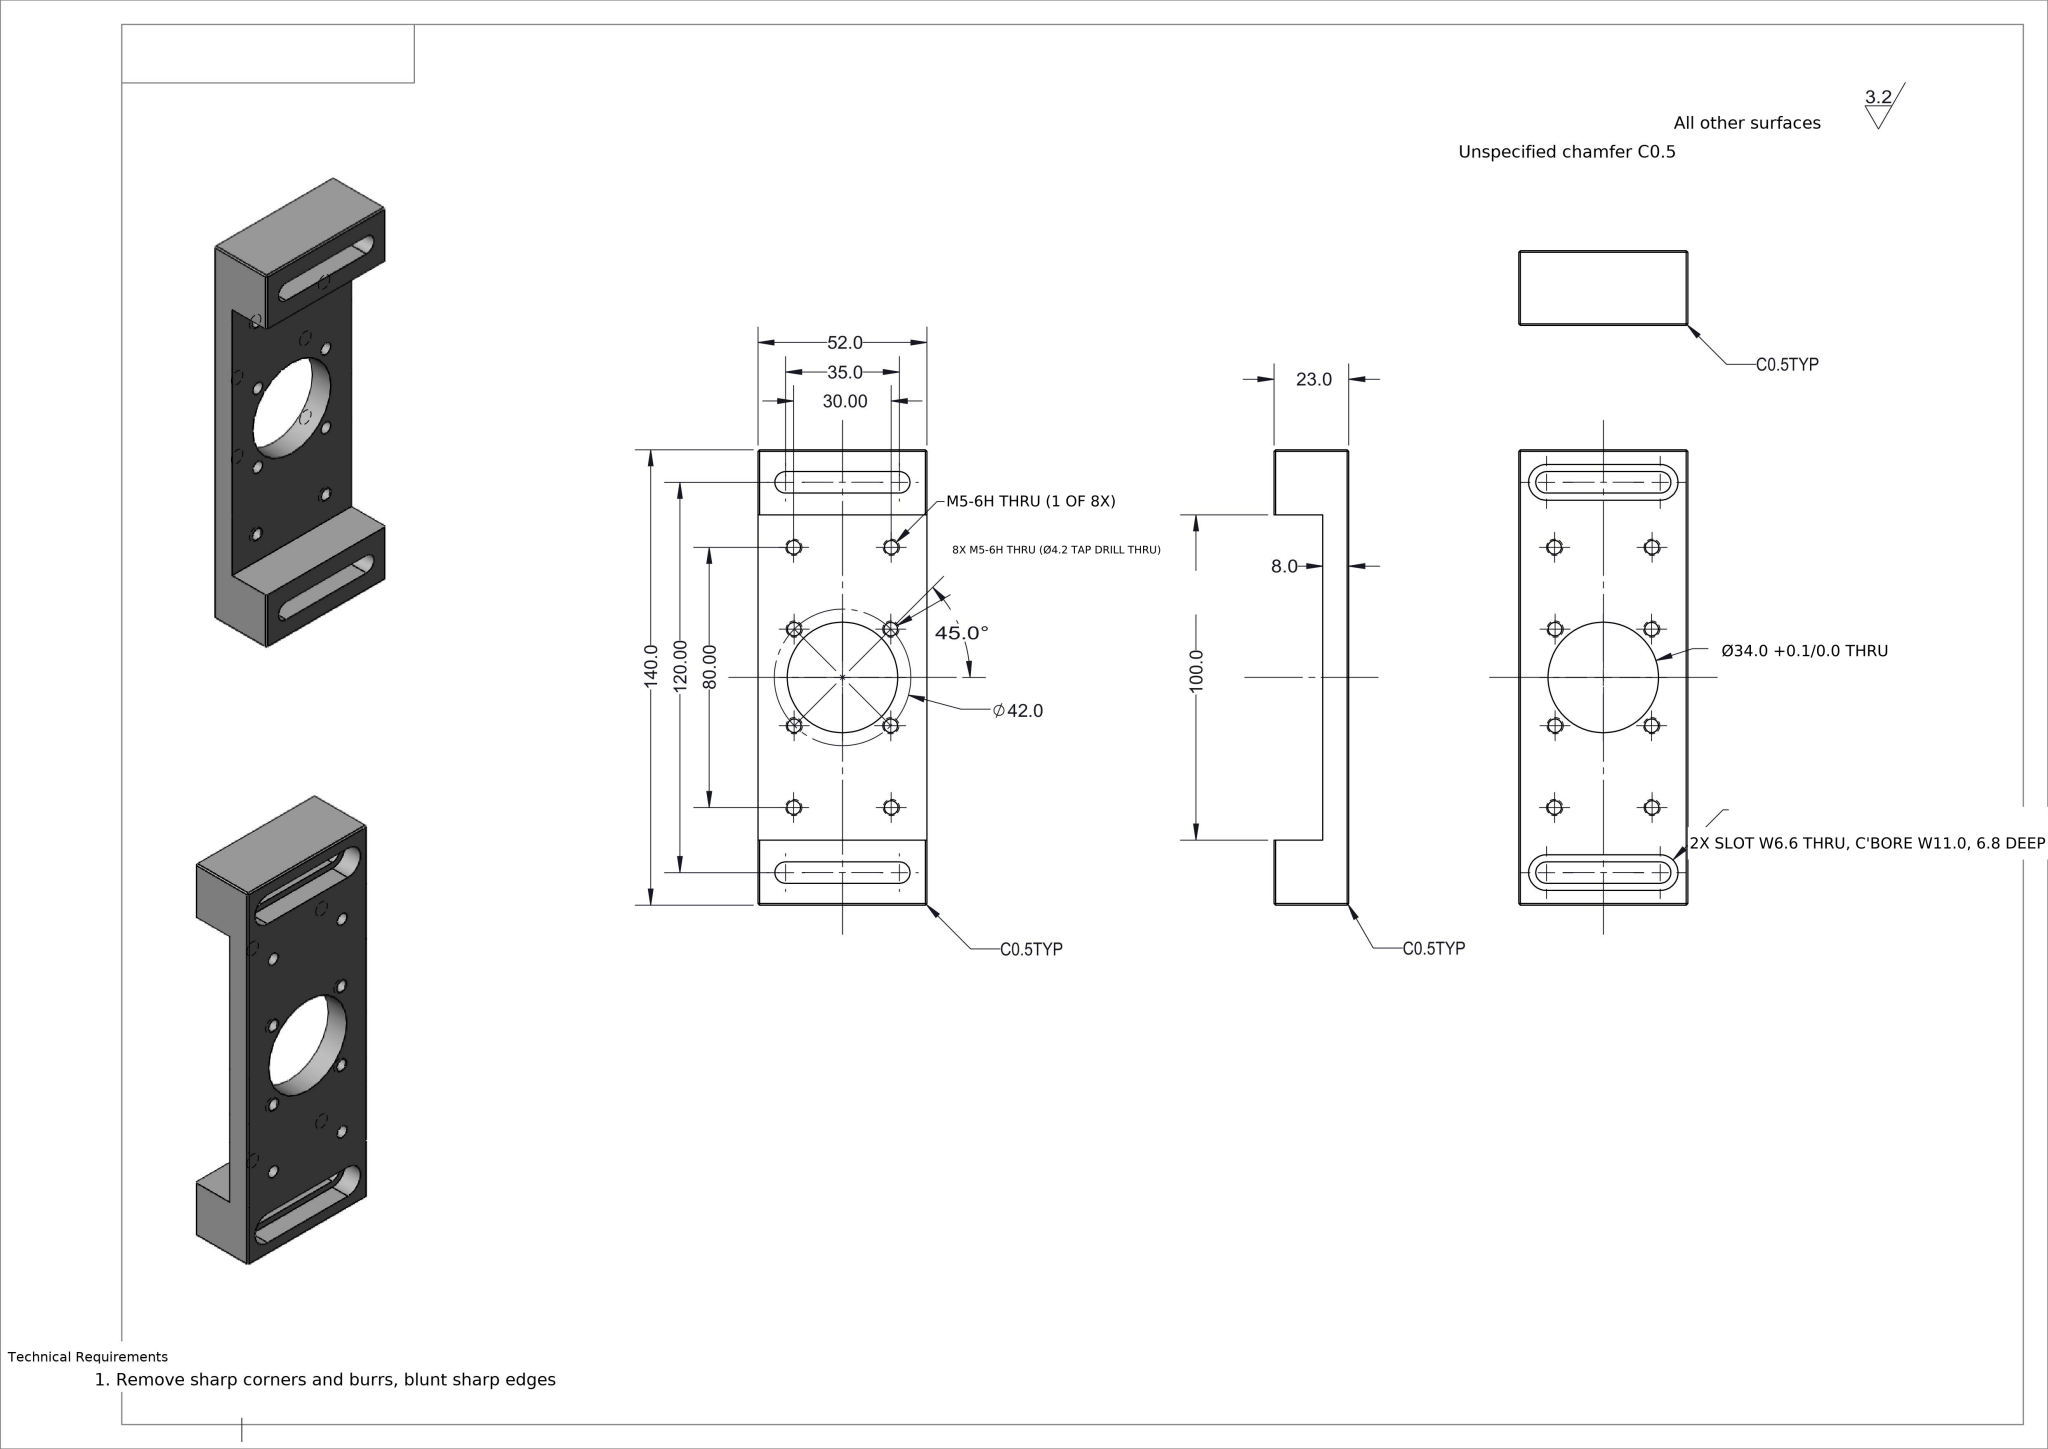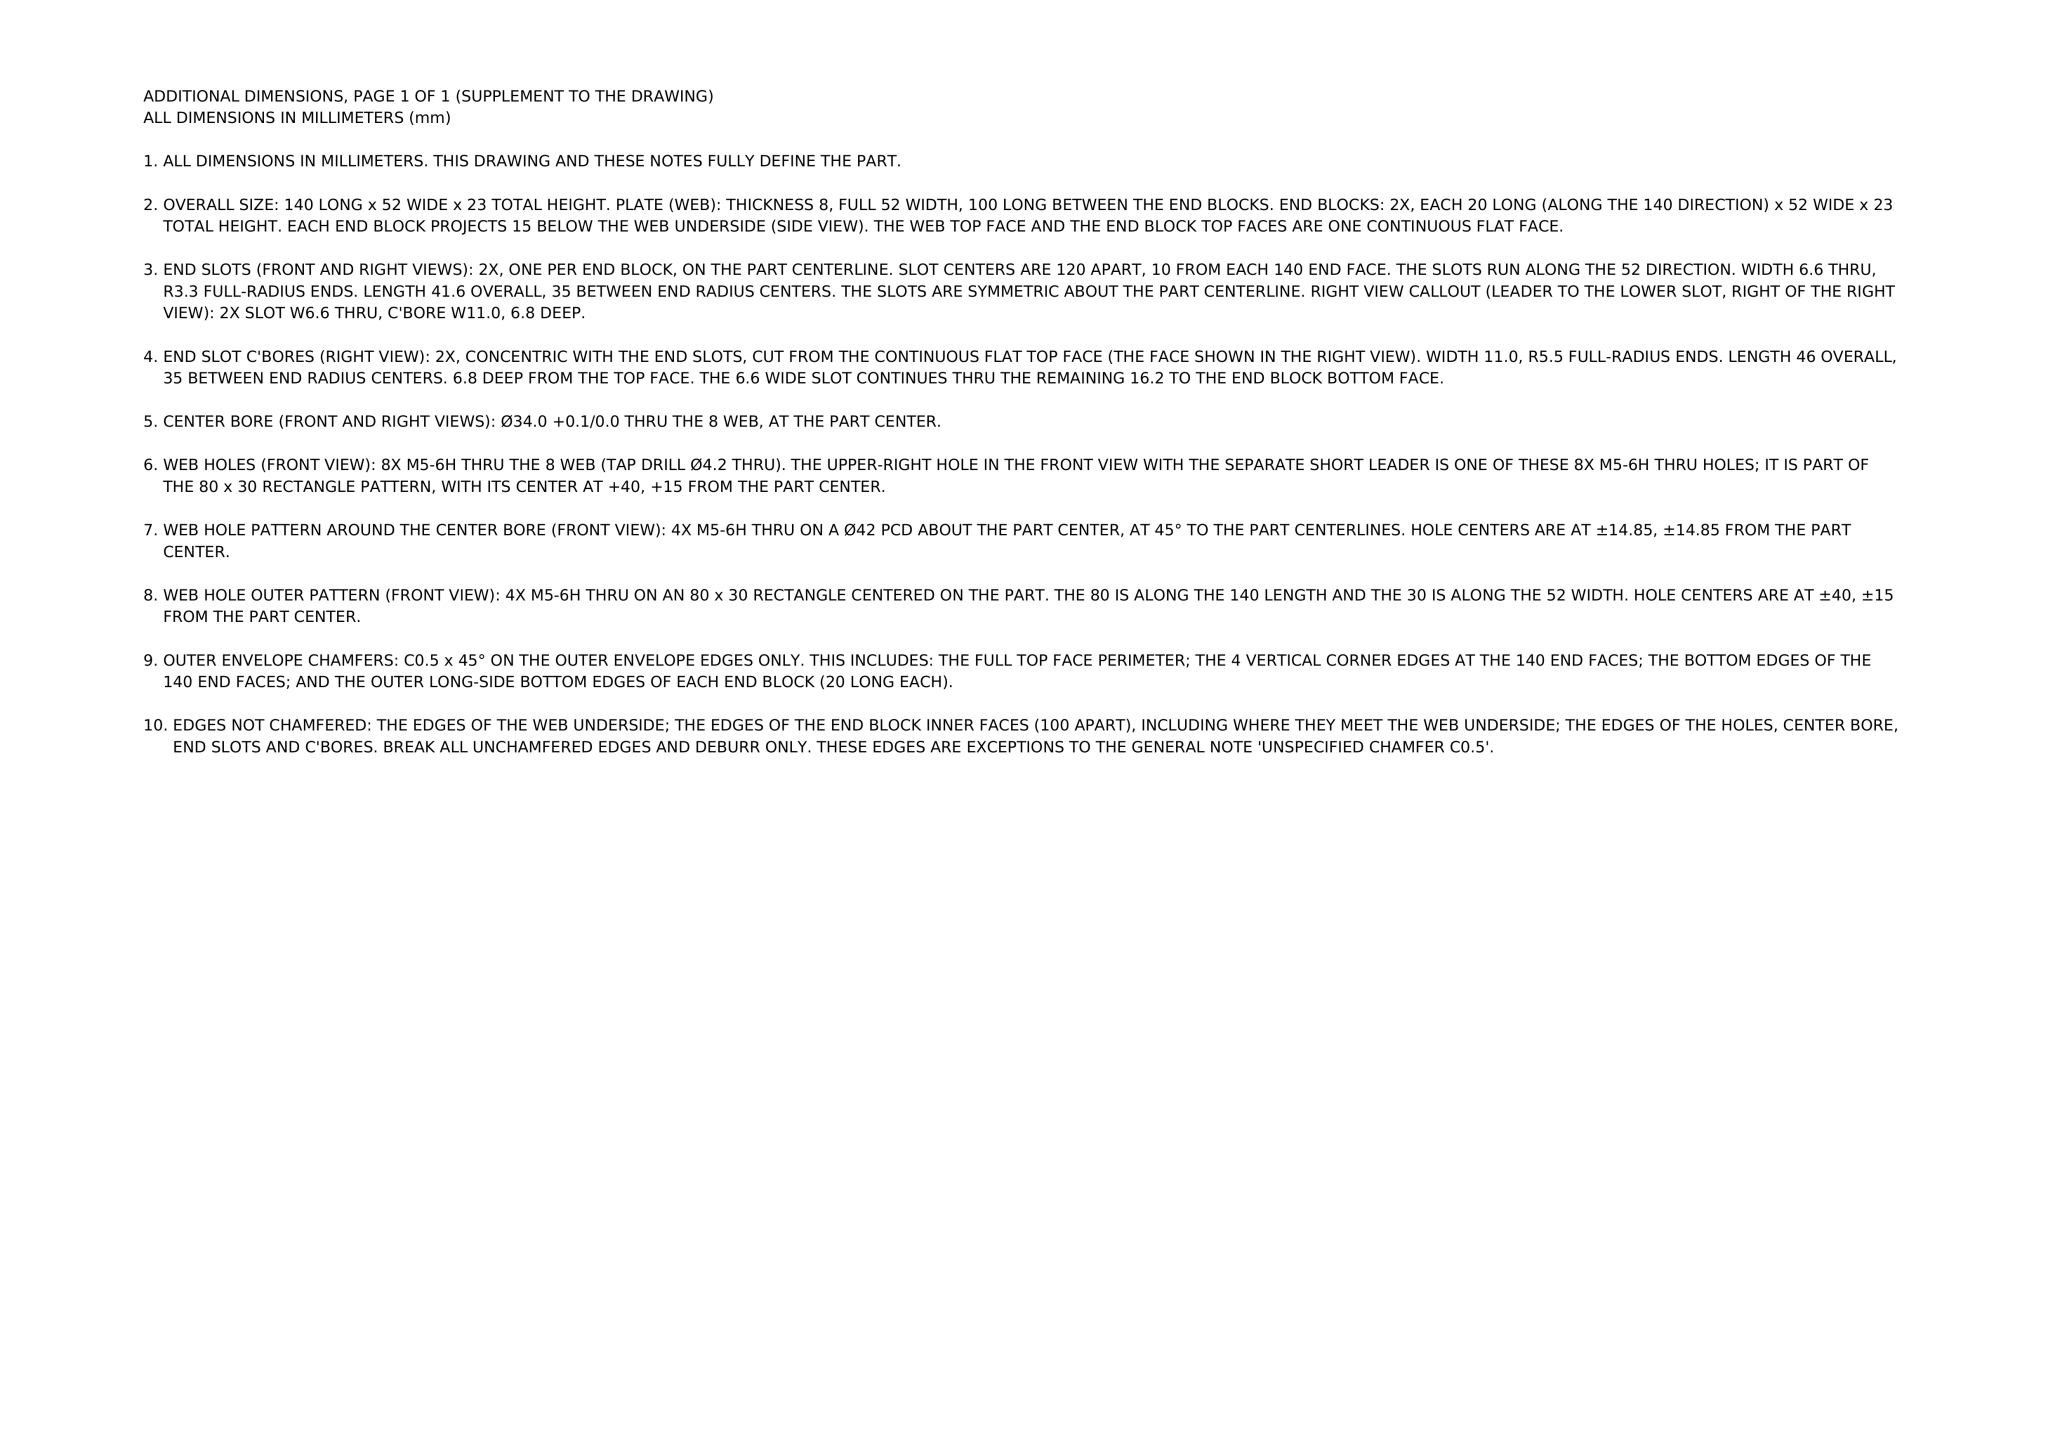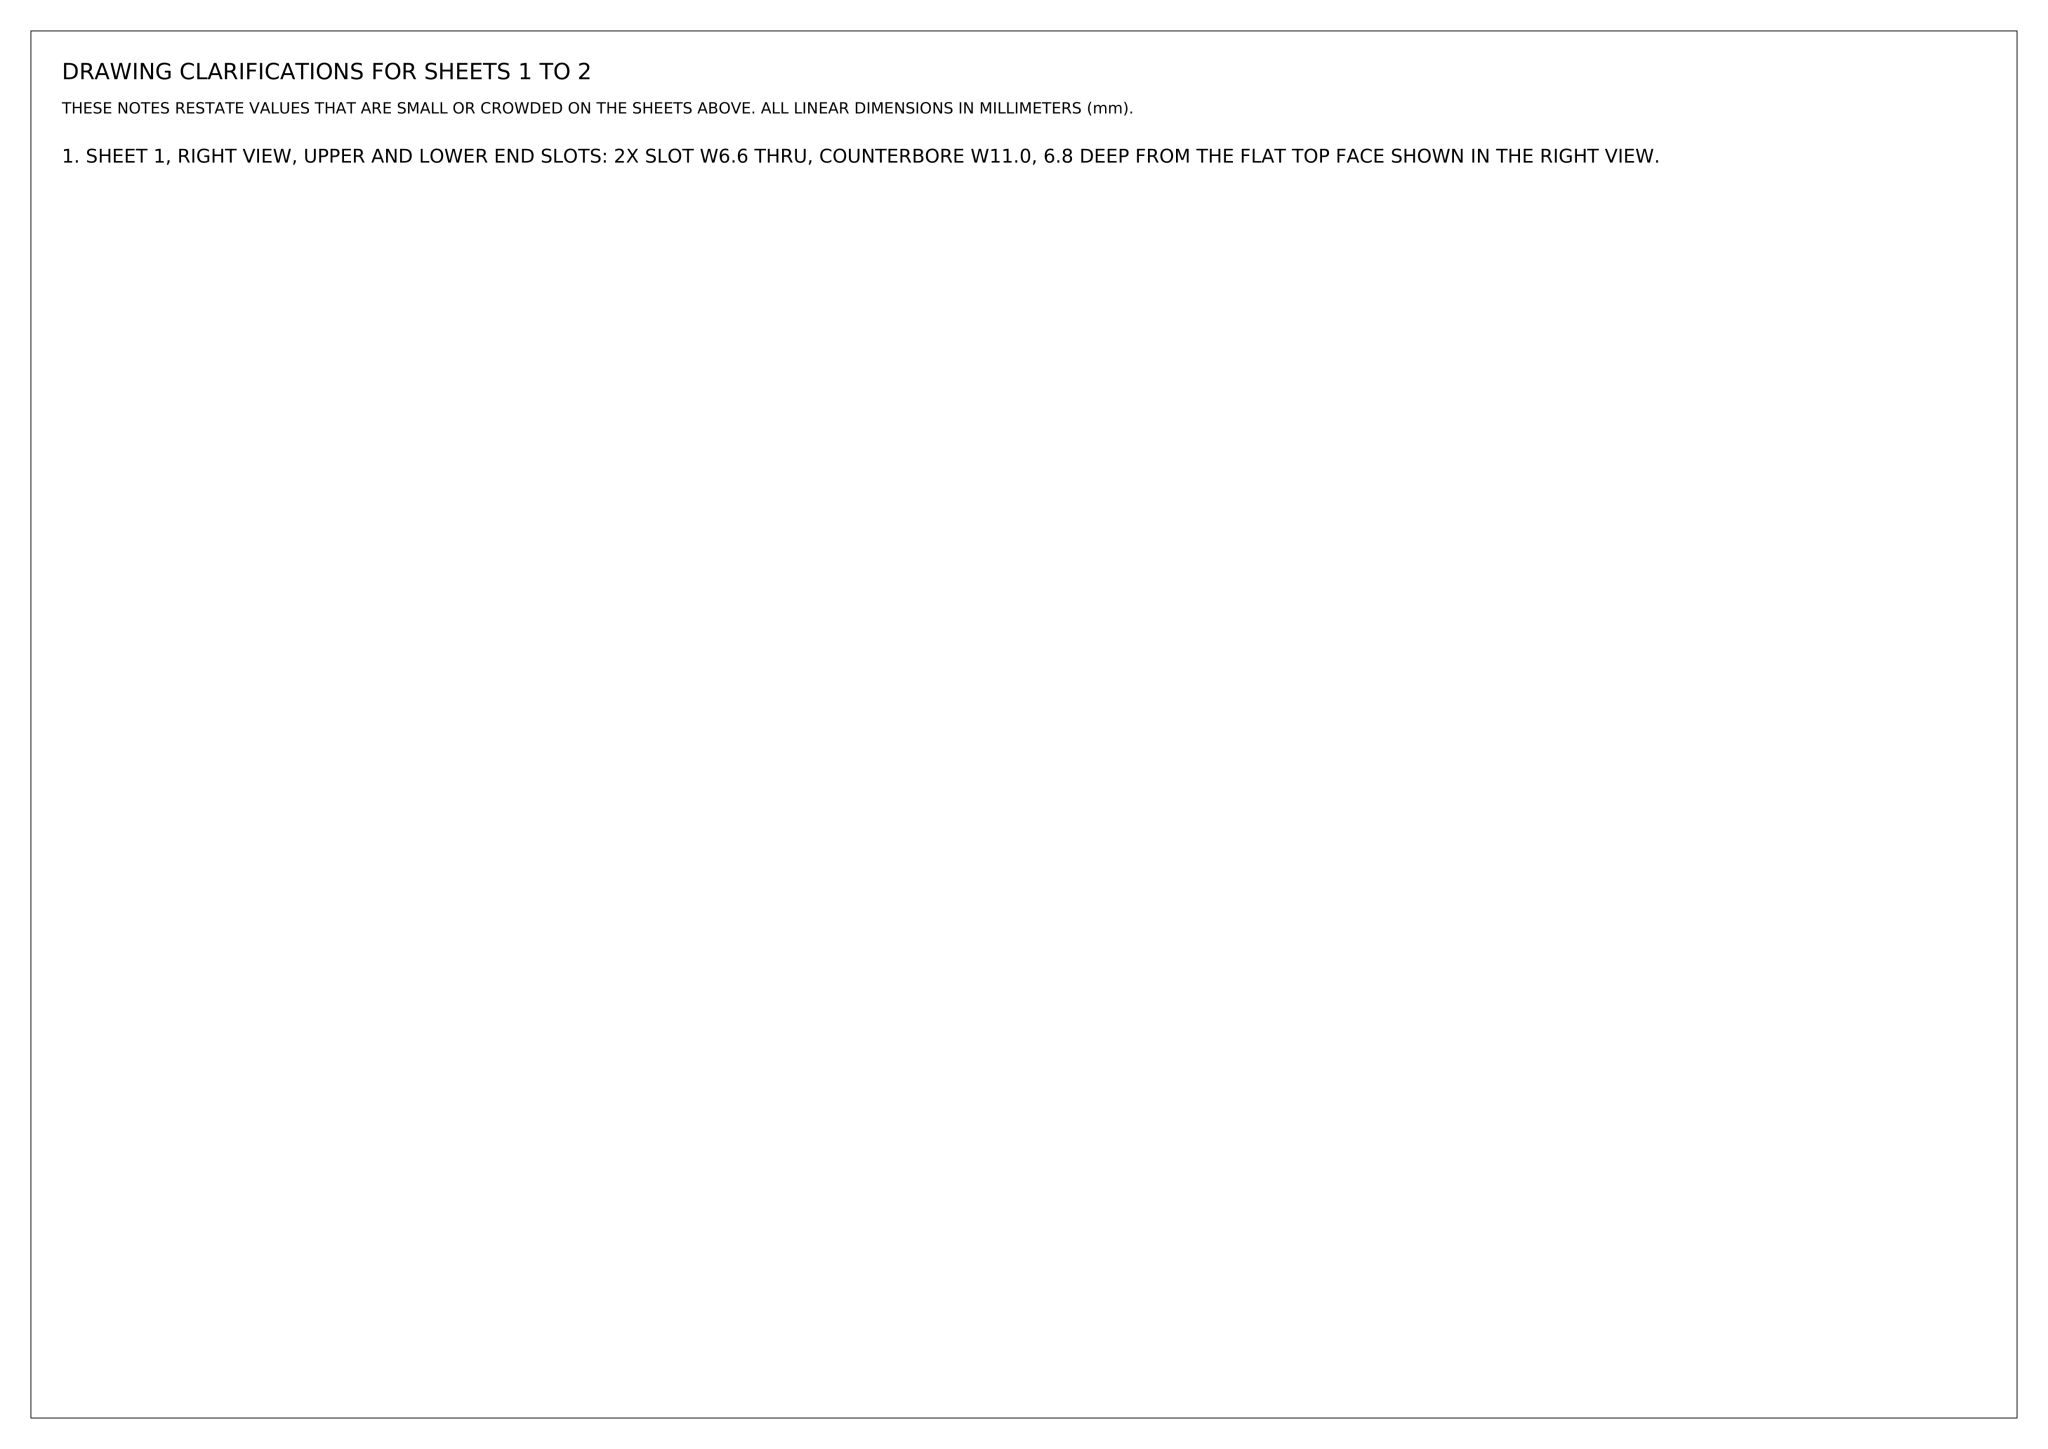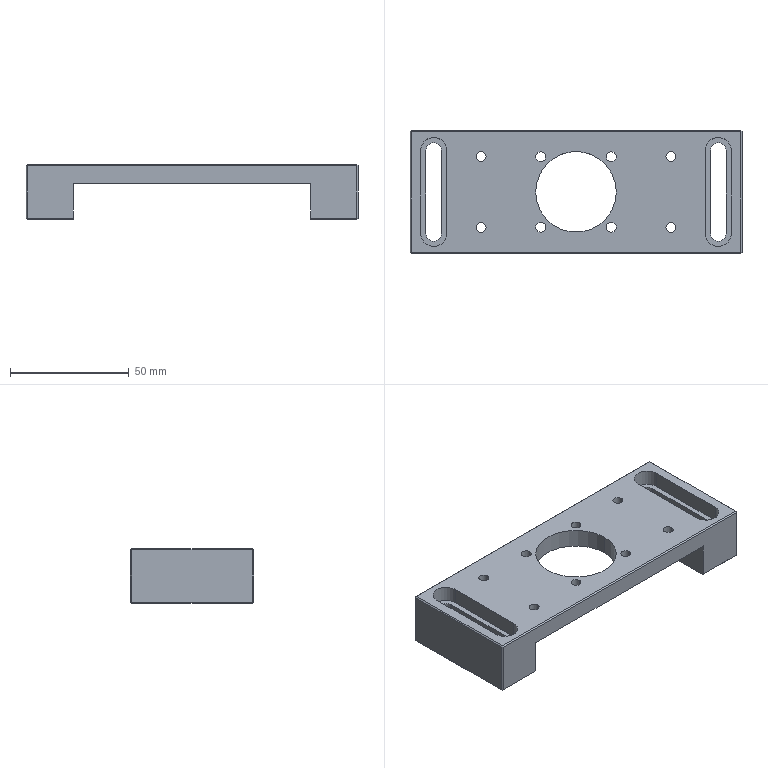Part | NX | mm | 1 solid | 68 faces | box 140 x 52 x 23 mm | volume 66087 mm3 | plane 42 | cylinder 26 | commonest cylinder face diameters 4.2 x16 6.6 x4 11 x4 34 x2